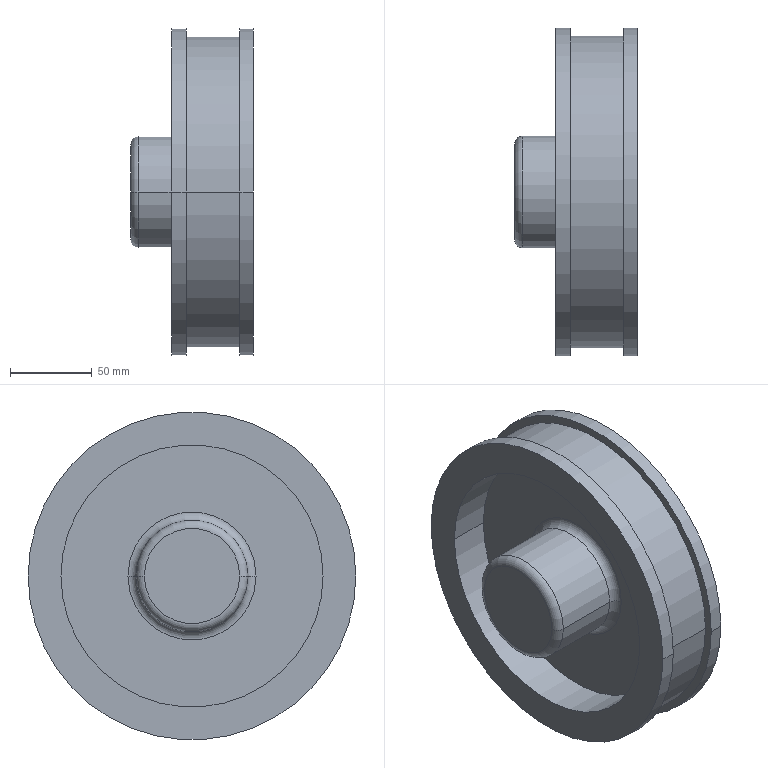Component | SolidWorks | AxisHead-1 | 1 solid | 23 faces | box 75 x 200 x 200 mm | volume 949663 mm3 | cylinder 12 | plane 7 | torus 4 | commonest cylinder face diameters 200 x4 160 x4 190 x2 68.235 x2
build123d program:
from build123d import *


with BuildPart() as part:
    # Sketch1 → Revolve1 (revolve)
    with BuildSketch(Plane.XZ, mode=Mode.PRIVATE) as revolve1_sk:
        with BuildLine():
            Line((80, 0.4717), (0, 0.4717))
            Line((0, 0.4717), (0, -64.528))
            Line((0, -64.528), (29.118, -64.528))
            ThreePointArc((29.118, -64.528), (32.653, -63.064), (34.118, -59.528))
            Line((34.118, -59.528), (34.118, -19.528))
            ThreePointArc((34.118, -19.528), (35.582, -15.993), (39.118, -14.528))
            Line((39.118, -14.528), (80, -14.528))
            Line((80, -14.528), (80, -39.528))
            Line((80, -39.528), (100, -39.528))
            Line((100, -39.528), (100, -30.551))
            Line((100, -30.551), (95, -30.551))
            Line((95, -30.551), (95, 2.206))
            Line((95, 2.206), (100, 2.206))
            Line((100, 2.206), (100, 10.472))
            Line((100, 10.472), (80, 10.472))
            Line((80, 10.472), (80, 0.4717))
        make_face()
    revolve(revolve1_sk.sketch.rotate(Axis((0, 0, 10.472), (0, 0, -1)), 180), axis=Axis((0, 0, 10.472), (0, 0, -1)))


solid = part.part

# Placed as in the assembly
solid = solid.moved(Location((-779.247, 870.769, 1116.347), (0, 90, 0)))
STEP:
#1=COLOUR_RGB('',0.7922,0.8196,0.9333);
#2=FILL_AREA_STYLE_COLOUR('',#1);
#3=FILL_AREA_STYLE('',(#2));
#4=SURFACE_STYLE_FILL_AREA(#3);
#5=SURFACE_SIDE_STYLE('',(#4));
#6=SURFACE_STYLE_USAGE(.BOTH.,#5);
#7=PRESENTATION_STYLE_ASSIGNMENT((#6));
#8=CARTESIAN_POINT('',(-30.267,30.345,43.951));
#9=VERTEX_POINT('',#8);
#10=CARTESIAN_POINT('',(-30.267,38.219,43.951));
#11=VERTEX_POINT('',#10);
#12=CARTESIAN_POINT('',(-30.267,34.282,43.951));
#13=DIRECTION('',(-1.,0.,0.));
#14=DIRECTION('',(0.,-1.,0.));
#15=AXIS2_PLACEMENT_3D('',#12,#13,#14);
#16=CIRCLE('',#15,3.937);
#17=EDGE_CURVE('',#9,#11,#16,.T.);
#18=ORIENTED_EDGE('',*,*,#17,.T.);
#19=CARTESIAN_POINT('',(-30.592,38.219,43.951));
#20=VERTEX_POINT('',#19);
#21=CARTESIAN_POINT('',(-30.267,38.219,43.951));
#22=DIRECTION('',(-1.,0.,0.));
#23=VECTOR('',#22,39.37);
#24=LINE('',#21,#23);
#25=EDGE_CURVE('',#11,#20,#24,.T.);
#26=ORIENTED_EDGE('',*,*,#25,.T.);
#27=CARTESIAN_POINT('',(-30.592,30.345,43.951));
#28=VERTEX_POINT('',#27);
#29=CARTESIAN_POINT('',(-30.592,34.282,43.951));
#30=DIRECTION('',(-1.,0.,0.));
#31=DIRECTION('',(0.,-1.,0.));
#32=AXIS2_PLACEMENT_3D('',#29,#30,#31);
#33=CIRCLE('',#32,3.937);
#34=EDGE_CURVE('',#28,#20,#33,.T.);
#35=ORIENTED_EDGE('',*,*,#34,.F.);
#36=CARTESIAN_POINT('',(-30.267,30.345,43.951));
#37=DIRECTION('',(-1.,0.,0.));
#38=VECTOR('',#37,39.37);
#39=LINE('',#36,#38);
#40=EDGE_CURVE('',#9,#28,#39,.T.);
#41=ORIENTED_EDGE('',*,*,#40,.F.);
#42=EDGE_LOOP('',(#18,#26,#35,#41));
#43=FACE_OUTER_BOUND('',#42,.T.);
#44=CARTESIAN_POINT('',(-30.267,34.282,43.951));
#45=DIRECTION('',(-1.,0.,0.));
#46=DIRECTION('',(0.,-1.,0.));
#47=AXIS2_PLACEMENT_3D('',#44,#45,#46);
#48=CYLINDRICAL_SURFACE('',#47,3.937);
#49=ADVANCED_FACE('',(#43),#48,.T.);
#50=CARTESIAN_POINT('',(-30.592,30.542,43.951));
#51=VERTEX_POINT('',#50);
#52=CARTESIAN_POINT('',(-30.592,38.022,43.951));
#53=VERTEX_POINT('',#52);
#54=CARTESIAN_POINT('',(-30.592,34.282,43.951));
#55=DIRECTION('',(-1.,0.,0.));
#56=DIRECTION('',(0.,-1.,0.));
#57=AXIS2_PLACEMENT_3D('',#54,#55,#56);
#58=CIRCLE('',#57,3.74);
#59=EDGE_CURVE('',#51,#53,#58,.T.);
#60=ORIENTED_EDGE('',*,*,#59,.T.);
#61=CARTESIAN_POINT('',(-31.882,38.022,43.951));
#62=VERTEX_POINT('',#61);
#63=CARTESIAN_POINT('',(-30.267,38.022,43.951));
#64=DIRECTION('',(-1.,0.,0.));
#65=VECTOR('',#64,39.37);
#66=LINE('',#63,#65);
#67=EDGE_CURVE('',#53,#62,#66,.T.);
#68=ORIENTED_EDGE('',*,*,#67,.T.);
#69=CARTESIAN_POINT('',(-31.882,30.542,43.951));
#70=VERTEX_POINT('',#69);
#71=CARTESIAN_POINT('',(-31.882,34.282,43.951));
#72=DIRECTION('',(-1.,0.,0.));
#73=DIRECTION('',(0.,-1.,0.));
#74=AXIS2_PLACEMENT_3D('',#71,#72,#73);
#75=CIRCLE('',#74,3.74);
#76=EDGE_CURVE('',#70,#62,#75,.T.);
#77=ORIENTED_EDGE('',*,*,#76,.F.);
#78=CARTESIAN_POINT('',(-30.267,30.542,43.951));
#79=DIRECTION('',(-1.,0.,0.));
#80=VECTOR('',#79,39.37);
#81=LINE('',#78,#80);
#82=EDGE_CURVE('',#51,#70,#81,.T.);
#83=ORIENTED_EDGE('',*,*,#82,.F.);
#84=EDGE_LOOP('',(#60,#68,#77,#83));
#85=FACE_OUTER_BOUND('',#84,.T.);
#86=CARTESIAN_POINT('',(-30.267,34.282,43.951));
#87=DIRECTION('',(-1.,0.,0.));
#88=DIRECTION('',(0.,-1.,0.));
#89=AXIS2_PLACEMENT_3D('',#86,#87,#88);
#90=CYLINDRICAL_SURFACE('',#89,3.74);
#91=ADVANCED_FACE('',(#85),#90,.T.);
#92=CARTESIAN_POINT('',(-31.882,30.345,43.951));
#93=VERTEX_POINT('',#92);
#94=CARTESIAN_POINT('',(-31.882,38.219,43.951));
#95=VERTEX_POINT('',#94);
#96=CARTESIAN_POINT('',(-31.882,34.282,43.951));
#97=DIRECTION('',(-1.,0.,0.));
#98=DIRECTION('',(0.,-1.,0.));
#99=AXIS2_PLACEMENT_3D('',#96,#97,#98);
#100=CIRCLE('',#99,3.937);
#101=EDGE_CURVE('',#93,#95,#100,.T.);
#102=ORIENTED_EDGE('',*,*,#101,.T.);
#103=CARTESIAN_POINT('',(-32.235,38.219,43.951));
#104=VERTEX_POINT('',#103);
#105=CARTESIAN_POINT('',(-30.267,38.219,43.951));
#106=DIRECTION('',(-1.,0.,0.));
#107=VECTOR('',#106,39.37);
#108=LINE('',#105,#107);
#109=EDGE_CURVE('',#95,#104,#108,.T.);
#110=ORIENTED_EDGE('',*,*,#109,.T.);
#111=CARTESIAN_POINT('',(-32.235,30.345,43.951));
#112=VERTEX_POINT('',#111);
#113=CARTESIAN_POINT('',(-32.235,34.282,43.951));
#114=DIRECTION('',(-1.,0.,0.));
#115=DIRECTION('',(0.,-1.,0.));
#116=AXIS2_PLACEMENT_3D('',#113,#114,#115);
#117=CIRCLE('',#116,3.937);
#118=EDGE_CURVE('',#112,#104,#117,.T.);
#119=ORIENTED_EDGE('',*,*,#118,.F.);
#120=CARTESIAN_POINT('',(-30.267,30.345,43.951));
#121=DIRECTION('',(-1.,0.,0.));
#122=VECTOR('',#121,39.37);
#123=LINE('',#120,#122);
#124=EDGE_CURVE('',#93,#112,#123,.T.);
#125=ORIENTED_EDGE('',*,*,#124,.F.);
#126=EDGE_LOOP('',(#102,#110,#119,#125));
#127=FACE_OUTER_BOUND('',#126,.T.);
#128=CARTESIAN_POINT('',(-30.267,34.282,43.951));
#129=DIRECTION('',(-1.,0.,0.));
#130=DIRECTION('',(0.,-1.,0.));
#131=AXIS2_PLACEMENT_3D('',#128,#129,#130);
#132=CYLINDRICAL_SURFACE('',#131,3.937);
#133=ADVANCED_FACE('',(#127),#132,.T.);
#134=CARTESIAN_POINT('',(-31.251,37.432,43.951));
#135=VERTEX_POINT('',#134);
#136=CARTESIAN_POINT('',(-31.251,31.133,43.951));
#137=VERTEX_POINT('',#136);
#138=CARTESIAN_POINT('',(-31.251,34.282,43.951));
#139=DIRECTION('',(-1.,0.,0.));
#140=DIRECTION('',(0.,-1.,0.));
#141=AXIS2_PLACEMENT_3D('',#138,#139,#140);
#142=CIRCLE('',#141,3.15);
#143=EDGE_CURVE('',#135,#137,#142,.T.);
#144=ORIENTED_EDGE('',*,*,#143,.F.);
#145=CARTESIAN_POINT('',(-32.235,37.432,43.951));
#146=VERTEX_POINT('',#145);
#147=CARTESIAN_POINT('',(-30.267,37.432,43.951));
#148=DIRECTION('',(-1.,0.,0.));
#149=VECTOR('',#148,39.37);
#150=LINE('',#147,#149);
#151=EDGE_CURVE('',#135,#146,#150,.T.);
#152=ORIENTED_EDGE('',*,*,#151,.T.);
#153=CARTESIAN_POINT('',(-32.235,31.133,43.951));
#154=VERTEX_POINT('',#153);
#155=CARTESIAN_POINT('',(-32.235,34.282,43.951));
#156=DIRECTION('',(-1.,0.,0.));
#157=DIRECTION('',(0.,-1.,0.));
#158=AXIS2_PLACEMENT_3D('',#155,#156,#157);
#159=CIRCLE('',#158,3.15);
#160=EDGE_CURVE('',#146,#154,#159,.T.);
#161=ORIENTED_EDGE('',*,*,#160,.T.);
#162=CARTESIAN_POINT('',(-30.267,31.133,43.951));
#163=DIRECTION('',(-1.,0.,0.));
#164=VECTOR('',#163,39.37);
#165=LINE('',#162,#164);
#166=EDGE_CURVE('',#137,#154,#165,.T.);
#167=ORIENTED_EDGE('',*,*,#166,.F.);
#168=EDGE_LOOP('',(#144,#152,#161,#167));
#169=FACE_OUTER_BOUND('',#168,.T.);
#170=CARTESIAN_POINT('',(-30.267,34.282,43.951));
#171=DIRECTION('',(-1.,0.,0.));
#172=DIRECTION('',(0.,-1.,0.));
#173=AXIS2_PLACEMENT_3D('',#170,#171,#172);
#174=CYLINDRICAL_SURFACE('',#173,3.15);
#175=ADVANCED_FACE('',(#169),#174,.F.);
#176=CARTESIAN_POINT('',(-31.448,35.625,43.951));
#177=VERTEX_POINT('',#176);
#178=CARTESIAN_POINT('',(-31.448,32.939,43.951));
#179=VERTEX_POINT('',#178);
#180=CARTESIAN_POINT('',(-31.448,34.282,43.951));
#181=DIRECTION('',(-1.,0.,0.));
#182=DIRECTION('',(0.,-1.,0.));
#183=AXIS2_PLACEMENT_3D('',#180,#181,#182);
#184=CIRCLE('',#183,1.343);
#185=EDGE_CURVE('',#177,#179,#184,.T.);
#186=ORIENTED_EDGE('',*,*,#185,.F.);
#187=CARTESIAN_POINT('',(-31.251,35.822,43.951));
#188=VERTEX_POINT('',#187);
#189=CARTESIAN_POINT('',(-31.448,35.822,43.951));
#190=DIRECTION('',(0.,-0.,1.));
#191=DIRECTION('',(0.,-1.,0.));
#192=AXIS2_PLACEMENT_3D('',#189,#190,#191);
#193=CIRCLE('',#192,0.1969);
#194=EDGE_CURVE('',#177,#188,#193,.T.);
#195=ORIENTED_EDGE('',*,*,#194,.T.);
#196=CARTESIAN_POINT('',(-31.251,32.742,43.951));
#197=VERTEX_POINT('',#196);
#198=CARTESIAN_POINT('',(-31.251,34.282,43.951));
#199=DIRECTION('',(-1.,0.,0.));
#200=DIRECTION('',(0.,-1.,0.));
#201=AXIS2_PLACEMENT_3D('',#198,#199,#200);
#202=CIRCLE('',#201,1.54);
#203=EDGE_CURVE('',#188,#197,#202,.T.);
#204=ORIENTED_EDGE('',*,*,#203,.T.);
#205=CARTESIAN_POINT('',(-31.448,32.742,43.951));
#206=DIRECTION('',(0.,0.,-1.));
#207=DIRECTION('',(-1.,0.,0.));
#208=AXIS2_PLACEMENT_3D('',#205,#206,#207);
#209=CIRCLE('',#208,0.1969);
#210=EDGE_CURVE('',#179,#197,#209,.T.);
#211=ORIENTED_EDGE('',*,*,#210,.F.);
#212=EDGE_LOOP('',(#186,#195,#204,#211));
#213=FACE_OUTER_BOUND('',#212,.T.);
#214=CARTESIAN_POINT('',(-31.448,34.282,43.951));
#215=DIRECTION('',(-1.,0.,0.));
#216=DIRECTION('',(0.,-1.,0.));
#217=AXIS2_PLACEMENT_3D('',#214,#215,#216);
#218=TOROIDAL_SURFACE('',#217,1.54,0.1969);
#219=ADVANCED_FACE('',(#213),#218,.F.);
#220=CARTESIAN_POINT('',(-31.448,34.282,43.951));
#221=DIRECTION('',(-1.,0.,0.));
#222=DIRECTION('',(0.,-1.,0.));
#223=AXIS2_PLACEMENT_3D('',#220,#221,#222);
#224=CIRCLE('',#223,1.343);
#225=EDGE_CURVE('',#179,#177,#224,.T.);
#226=ORIENTED_EDGE('',*,*,#225,.T.);
#227=CARTESIAN_POINT('',(-33.023,35.625,43.951));
#228=VERTEX_POINT('',#227);
#229=CARTESIAN_POINT('',(-30.267,35.625,43.951));
#230=DIRECTION('',(-1.,0.,0.));
#231=VECTOR('',#230,39.37);
#232=LINE('',#229,#231);
#233=EDGE_CURVE('',#177,#228,#232,.T.);
#234=ORIENTED_EDGE('',*,*,#233,.T.);
#235=CARTESIAN_POINT('',(-33.023,32.939,43.951));
#236=VERTEX_POINT('',#235);
#237=CARTESIAN_POINT('',(-33.023,34.282,43.951));
#238=DIRECTION('',(-1.,0.,0.));
#239=DIRECTION('',(0.,-1.,0.));
#240=AXIS2_PLACEMENT_3D('',#237,#238,#239);
#241=CIRCLE('',#240,1.343);
#242=EDGE_CURVE('',#236,#228,#241,.T.);
#243=ORIENTED_EDGE('',*,*,#242,.F.);
#244=CARTESIAN_POINT('',(-30.267,32.939,43.951));
#245=DIRECTION('',(-1.,0.,0.));
#246=VECTOR('',#245,39.37);
#247=LINE('',#244,#246);
#248=EDGE_CURVE('',#179,#236,#247,.T.);
#249=ORIENTED_EDGE('',*,*,#248,.F.);
#250=EDGE_LOOP('',(#226,#234,#243,#249));
#251=FACE_OUTER_BOUND('',#250,.T.);
#252=CARTESIAN_POINT('',(-30.267,34.282,43.951));
#253=DIRECTION('',(-1.,0.,0.));
#254=DIRECTION('',(0.,-1.,0.));
#255=AXIS2_PLACEMENT_3D('',#252,#253,#254);
#256=CYLINDRICAL_SURFACE('',#255,1.343);
#257=ADVANCED_FACE('',(#251),#256,.T.);
#258=ORIENTED_EDGE('',*,*,#242,.T.);
#259=CARTESIAN_POINT('',(-33.219,35.429,43.951));
#260=VERTEX_POINT('',#259);
#261=CARTESIAN_POINT('',(-33.023,35.429,43.951));
#262=DIRECTION('',(0.,-0.,1.));
#263=DIRECTION('',(0.,-1.,0.));
#264=AXIS2_PLACEMENT_3D('',#261,#262,#263);
#265=CIRCLE('',#264,0.1969);
#266=EDGE_CURVE('',#228,#260,#265,.T.);
#267=ORIENTED_EDGE('',*,*,#266,.T.);
#268=CARTESIAN_POINT('',(-33.219,33.136,43.951));
#269=VERTEX_POINT('',#268);
#270=CARTESIAN_POINT('',(-33.219,34.282,43.951));
#271=DIRECTION('',(-1.,0.,0.));
#272=DIRECTION('',(0.,-1.,0.));
#273=AXIS2_PLACEMENT_3D('',#270,#271,#272);
#274=CIRCLE('',#273,1.146);
#275=EDGE_CURVE('',#269,#260,#274,.T.);
#276=ORIENTED_EDGE('',*,*,#275,.F.);
#277=CARTESIAN_POINT('',(-33.023,33.136,43.951));
#278=DIRECTION('',(0.,0.,-1.));
#279=DIRECTION('',(-1.,0.,0.));
#280=AXIS2_PLACEMENT_3D('',#277,#278,#279);
#281=CIRCLE('',#280,0.1969);
#282=EDGE_CURVE('',#236,#269,#281,.T.);
#283=ORIENTED_EDGE('',*,*,#282,.F.);
#284=EDGE_LOOP('',(#258,#267,#276,#283));
#285=FACE_OUTER_BOUND('',#284,.T.);
#286=CARTESIAN_POINT('',(-33.023,34.282,43.951));
#287=DIRECTION('',(-1.,0.,0.));
#288=DIRECTION('',(0.,-1.,0.));
#289=AXIS2_PLACEMENT_3D('',#286,#287,#288);
#290=TOROIDAL_SURFACE('',#289,1.146,0.1969);
#291=ADVANCED_FACE('',(#285),#290,.T.);
#292=CARTESIAN_POINT('',(-30.267,37.432,43.951));
#293=VERTEX_POINT('',#292);
#294=CARTESIAN_POINT('',(-30.267,31.133,43.951));
#295=VERTEX_POINT('',#294);
#296=CARTESIAN_POINT('',(-30.267,34.282,43.951));
#297=DIRECTION('',(-1.,0.,0.));
#298=DIRECTION('',(0.,-1.,0.));
#299=AXIS2_PLACEMENT_3D('',#296,#297,#298);
#300=CIRCLE('',#299,3.15);
#301=EDGE_CURVE('',#293,#295,#300,.T.);
#302=ORIENTED_EDGE('',*,*,#301,.F.);
#303=CARTESIAN_POINT('',(-30.66,37.432,43.951));
#304=VERTEX_POINT('',#303);
#305=CARTESIAN_POINT('',(-30.267,37.432,43.951));
#306=DIRECTION('',(-1.,0.,0.));
#307=VECTOR('',#306,39.37);
#308=LINE('',#305,#307);
#309=EDGE_CURVE('',#293,#304,#308,.T.);
#310=ORIENTED_EDGE('',*,*,#309,.T.);
#311=CARTESIAN_POINT('',(-30.66,31.133,43.951));
#312=VERTEX_POINT('',#311);
#313=CARTESIAN_POINT('',(-30.66,34.282,43.951));
#314=DIRECTION('',(-1.,0.,0.));
#315=DIRECTION('',(0.,-1.,0.));
#316=AXIS2_PLACEMENT_3D('',#313,#314,#315);
#317=CIRCLE('',#316,3.15);
#318=EDGE_CURVE('',#304,#312,#317,.T.);
#319=ORIENTED_EDGE('',*,*,#318,.T.);
#320=CARTESIAN_POINT('',(-30.267,31.133,43.951));
#321=DIRECTION('',(-1.,0.,0.));
#322=VECTOR('',#321,39.37);
#323=LINE('',#320,#322);
#324=EDGE_CURVE('',#295,#312,#323,.T.);
#325=ORIENTED_EDGE('',*,*,#324,.F.);
#326=EDGE_LOOP('',(#302,#310,#319,#325));
#327=FACE_OUTER_BOUND('',#326,.T.);
#328=CARTESIAN_POINT('',(-30.267,34.282,43.951));
#329=DIRECTION('',(-1.,0.,0.));
#330=DIRECTION('',(0.,-1.,0.));
#331=AXIS2_PLACEMENT_3D('',#328,#329,#330);
#332=CYLINDRICAL_SURFACE('',#331,3.15);
#333=ADVANCED_FACE('',(#327),#332,.F.);
#334=ORIENTED_EDGE('',*,*,#309,.F.);
#335=CARTESIAN_POINT('',(-30.267,34.282,43.951));
#336=DIRECTION('',(-1.,0.,0.));
#337=DIRECTION('',(0.,-1.,0.));
#338=AXIS2_PLACEMENT_3D('',#335,#336,#337);
#339=CIRCLE('',#338,3.15);
#340=EDGE_CURVE('',#295,#293,#339,.T.);
#341=ORIENTED_EDGE('',*,*,#340,.F.);
#342=ORIENTED_EDGE('',*,*,#324,.T.);
#343=CARTESIAN_POINT('',(-30.66,34.282,43.951));
#344=DIRECTION('',(-1.,0.,0.));
#345=DIRECTION('',(0.,-1.,0.));
#346=AXIS2_PLACEMENT_3D('',#343,#344,#345);
#347=CIRCLE('',#346,3.15);
#348=EDGE_CURVE('',#312,#304,#347,.T.);
#349=ORIENTED_EDGE('',*,*,#348,.T.);
#350=EDGE_LOOP('',(#334,#341,#342,#349));
#351=FACE_OUTER_BOUND('',#350,.T.);
#352=CARTESIAN_POINT('',(-30.267,34.282,43.951));
#353=DIRECTION('',(-1.,0.,0.));
#354=DIRECTION('',(0.,-1.,0.));
#355=AXIS2_PLACEMENT_3D('',#352,#353,#354);
#356=CYLINDRICAL_SURFACE('',#355,3.15);
#357=ADVANCED_FACE('',(#351),#356,.F.);
#358=ORIENTED_EDGE('',*,*,#348,.F.);
#359=ORIENTED_EDGE('',*,*,#318,.F.);
#360=EDGE_LOOP('',(#358,#359));
#361=FACE_OUTER_BOUND('',#360,.T.);
#362=CARTESIAN_POINT('',(-30.66,37.432,43.951));
#363=DIRECTION('',(1.,0.,0.));
#364=DIRECTION('',(0.,1.,0.));
#365=AXIS2_PLACEMENT_3D('',#362,#363,#364);
#366=PLANE('',#365);
#367=ADVANCED_FACE('',(#361),#366,.T.);
#368=ORIENTED_EDGE('',*,*,#275,.T.);
#369=CARTESIAN_POINT('',(-33.219,34.282,43.951));
#370=DIRECTION('',(-1.,0.,0.));
#371=DIRECTION('',(0.,-1.,0.));
#372=AXIS2_PLACEMENT_3D('',#369,#370,#371);
#373=CIRCLE('',#372,1.146);
#374=EDGE_CURVE('',#260,#269,#373,.T.);
#375=ORIENTED_EDGE('',*,*,#374,.T.);
#376=EDGE_LOOP('',(#368,#375));
#377=FACE_OUTER_BOUND('',#376,.T.);
#378=CARTESIAN_POINT('',(-33.219,34.282,43.951));
#379=DIRECTION('',(-1.,0.,0.));
#380=DIRECTION('',(0.,-1.,0.));
#381=AXIS2_PLACEMENT_3D('',#378,#379,#380);
#382=PLANE('',#381);
#383=ADVANCED_FACE('',(#377),#382,.T.);
#384=ORIENTED_EDGE('',*,*,#266,.F.);
#385=CARTESIAN_POINT('',(-33.023,34.282,43.951));
#386=DIRECTION('',(-1.,0.,0.));
#387=DIRECTION('',(0.,-1.,0.));
#388=AXIS2_PLACEMENT_3D('',#385,#386,#387);
#389=CIRCLE('',#388,1.343);
#390=EDGE_CURVE('',#228,#236,#389,.T.);
#391=ORIENTED_EDGE('',*,*,#390,.T.);
#392=ORIENTED_EDGE('',*,*,#282,.T.);
#393=ORIENTED_EDGE('',*,*,#374,.F.);
#394=EDGE_LOOP('',(#384,#391,#392,#393));
#395=FACE_OUTER_BOUND('',#394,.T.);
#396=CARTESIAN_POINT('',(-33.023,34.282,43.951));
#397=DIRECTION('',(-1.,0.,0.));
#398=DIRECTION('',(0.,-1.,0.));
#399=AXIS2_PLACEMENT_3D('',#396,#397,#398);
#400=TOROIDAL_SURFACE('',#399,1.146,0.1969);
#401=ADVANCED_FACE('',(#395),#400,.T.);
#402=ORIENTED_EDGE('',*,*,#233,.F.);
#403=ORIENTED_EDGE('',*,*,#185,.T.);
#404=ORIENTED_EDGE('',*,*,#248,.T.);
#405=ORIENTED_EDGE('',*,*,#390,.F.);
#406=EDGE_LOOP('',(#402,#403,#404,#405));
#407=FACE_OUTER_BOUND('',#406,.T.);
#408=CARTESIAN_POINT('',(-30.267,34.282,43.951));
#409=DIRECTION('',(-1.,0.,0.));
#410=DIRECTION('',(0.,-1.,0.));
#411=AXIS2_PLACEMENT_3D('',#408,#409,#410);
#412=CYLINDRICAL_SURFACE('',#411,1.343);
#413=ADVANCED_FACE('',(#407),#412,.T.);
#414=ORIENTED_EDGE('',*,*,#194,.F.);
#415=ORIENTED_EDGE('',*,*,#225,.F.);
#416=ORIENTED_EDGE('',*,*,#210,.T.);
#417=CARTESIAN_POINT('',(-31.251,34.282,43.951));
#418=DIRECTION('',(-1.,0.,0.));
#419=DIRECTION('',(0.,-1.,0.));
#420=AXIS2_PLACEMENT_3D('',#417,#418,#419);
#421=CIRCLE('',#420,1.54);
#422=EDGE_CURVE('',#197,#188,#421,.T.);
#423=ORIENTED_EDGE('',*,*,#422,.T.);
#424=EDGE_LOOP('',(#414,#415,#416,#423));
#425=FACE_OUTER_BOUND('',#424,.T.);
#426=CARTESIAN_POINT('',(-31.448,34.282,43.951));
#427=DIRECTION('',(-1.,0.,0.));
#428=DIRECTION('',(0.,-1.,0.));
#429=AXIS2_PLACEMENT_3D('',#426,#427,#428);
#430=TOROIDAL_SURFACE('',#429,1.54,0.1969);
#431=ADVANCED_FACE('',(#425),#430,.F.);
#432=CARTESIAN_POINT('',(-31.251,34.282,43.951));
#433=DIRECTION('',(-1.,0.,0.));
#434=DIRECTION('',(0.,-1.,0.));
#435=AXIS2_PLACEMENT_3D('',#432,#433,#434);
#436=CIRCLE('',#435,3.15);
#437=EDGE_CURVE('',#137,#135,#436,.T.);
#438=ORIENTED_EDGE('',*,*,#437,.T.);
#439=ORIENTED_EDGE('',*,*,#143,.T.);
#440=EDGE_LOOP('',(#438,#439));
#441=FACE_OUTER_BOUND('',#440,.T.);
#442=ORIENTED_EDGE('',*,*,#422,.F.);
#443=ORIENTED_EDGE('',*,*,#203,.F.);
#444=EDGE_LOOP('',(#442,#443));
#445=FACE_BOUND('',#444,.T.);
#446=CARTESIAN_POINT('',(-31.251,35.822,43.951));
#447=DIRECTION('',(-1.,0.,0.));
#448=DIRECTION('',(0.,-1.,0.));
#449=AXIS2_PLACEMENT_3D('',#446,#447,#448);
#450=PLANE('',#449);
#451=ADVANCED_FACE('',(#441,#445),#450,.T.);
#452=ORIENTED_EDGE('',*,*,#151,.F.);
#453=ORIENTED_EDGE('',*,*,#437,.F.);
#454=ORIENTED_EDGE('',*,*,#166,.T.);
#455=CARTESIAN_POINT('',(-32.235,34.282,43.951));
#456=DIRECTION('',(-1.,0.,0.));
#457=DIRECTION('',(0.,-1.,0.));
#458=AXIS2_PLACEMENT_3D('',#455,#456,#457);
#459=CIRCLE('',#458,3.15);
#460=EDGE_CURVE('',#154,#146,#459,.T.);
#461=ORIENTED_EDGE('',*,*,#460,.T.);
#462=EDGE_LOOP('',(#452,#453,#454,#461));
#463=FACE_OUTER_BOUND('',#462,.T.);
#464=CARTESIAN_POINT('',(-30.267,34.282,43.951));
#465=DIRECTION('',(-1.,0.,0.));
#466=DIRECTION('',(0.,-1.,0.));
#467=AXIS2_PLACEMENT_3D('',#464,#465,#466);
#468=CYLINDRICAL_SURFACE('',#467,3.15);
#469=ADVANCED_FACE('',(#463),#468,.F.);
#470=ORIENTED_EDGE('',*,*,#118,.T.);
#471=CARTESIAN_POINT('',(-32.235,34.282,43.951));
#472=DIRECTION('',(-1.,0.,0.));
#473=DIRECTION('',(0.,-1.,0.));
#474=AXIS2_PLACEMENT_3D('',#471,#472,#473);
#475=CIRCLE('',#474,3.937);
#476=EDGE_CURVE('',#104,#112,#475,.T.);
#477=ORIENTED_EDGE('',*,*,#476,.T.);
#478=EDGE_LOOP('',(#470,#477));
#479=FACE_OUTER_BOUND('',#478,.T.);
#480=ORIENTED_EDGE('',*,*,#460,.F.);
#481=ORIENTED_EDGE('',*,*,#160,.F.);
#482=EDGE_LOOP('',(#480,#481));
#483=FACE_BOUND('',#482,.T.);
#484=CARTESIAN_POINT('',(-32.235,37.432,43.951));
#485=DIRECTION('',(-1.,0.,0.));
#486=DIRECTION('',(0.,-1.,0.));
#487=AXIS2_PLACEMENT_3D('',#484,#485,#486);
#488=PLANE('',#487);
#489=ADVANCED_FACE('',(#479,#483),#488,.T.);
#490=ORIENTED_EDGE('',*,*,#109,.F.);
#491=CARTESIAN_POINT('',(-31.882,34.282,43.951));
#492=DIRECTION('',(-1.,0.,0.));
#493=DIRECTION('',(0.,-1.,0.));
#494=AXIS2_PLACEMENT_3D('',#491,#492,#493);
#495=CIRCLE('',#494,3.937);
#496=EDGE_CURVE('',#95,#93,#495,.T.);
#497=ORIENTED_EDGE('',*,*,#496,.T.);
#498=ORIENTED_EDGE('',*,*,#124,.T.);
#499=ORIENTED_EDGE('',*,*,#476,.F.);
#500=EDGE_LOOP('',(#490,#497,#498,#499));
#501=FACE_OUTER_BOUND('',#500,.T.);
#502=CARTESIAN_POINT('',(-30.267,34.282,43.951));
#503=DIRECTION('',(-1.,0.,0.));
#504=DIRECTION('',(0.,-1.,0.));
#505=AXIS2_PLACEMENT_3D('',#502,#503,#504);
#506=CYLINDRICAL_SURFACE('',#505,3.937);
#507=ADVANCED_FACE('',(#501),#506,.T.);
#508=ORIENTED_EDGE('',*,*,#76,.T.);
#509=CARTESIAN_POINT('',(-31.882,34.282,43.951));
#510=DIRECTION('',(-1.,0.,0.));
#511=DIRECTION('',(0.,-1.,0.));
#512=AXIS2_PLACEMENT_3D('',#509,#510,#511);
#513=CIRCLE('',#512,3.74);
#514=EDGE_CURVE('',#62,#70,#513,.T.);
#515=ORIENTED_EDGE('',*,*,#514,.T.);
#516=EDGE_LOOP('',(#508,#515));
#517=FACE_BOUND('',#516,.T.);
#518=ORIENTED_EDGE('',*,*,#101,.F.);
#519=ORIENTED_EDGE('',*,*,#496,.F.);
#520=EDGE_LOOP('',(#518,#519));
#521=FACE_OUTER_BOUND('',#520,.T.);
#522=CARTESIAN_POINT('',(-31.882,38.219,43.951));
#523=DIRECTION('',(1.,0.,0.));
#524=DIRECTION('',(0.,1.,0.));
#525=AXIS2_PLACEMENT_3D('',#522,#523,#524);
#526=PLANE('',#525);
#527=ADVANCED_FACE('',(#517,#521),#526,.T.);
#528=ORIENTED_EDGE('',*,*,#67,.F.);
#529=CARTESIAN_POINT('',(-30.592,34.282,43.951));
#530=DIRECTION('',(-1.,0.,0.));
#531=DIRECTION('',(0.,-1.,0.));
#532=AXIS2_PLACEMENT_3D('',#529,#530,#531);
#533=CIRCLE('',#532,3.74);
#534=EDGE_CURVE('',#53,#51,#533,.T.);
#535=ORIENTED_EDGE('',*,*,#534,.T.);
#536=ORIENTED_EDGE('',*,*,#82,.T.);
#537=ORIENTED_EDGE('',*,*,#514,.F.);
#538=EDGE_LOOP('',(#528,#535,#536,#537));
#539=FACE_OUTER_BOUND('',#538,.T.);
#540=CARTESIAN_POINT('',(-30.267,34.282,43.951));
#541=DIRECTION('',(-1.,0.,0.));
#542=DIRECTION('',(0.,-1.,0.));
#543=AXIS2_PLACEMENT_3D('',#540,#541,#542);
#544=CYLINDRICAL_SURFACE('',#543,3.74);
#545=ADVANCED_FACE('',(#539),#544,.T.);
#546=ORIENTED_EDGE('',*,*,#34,.T.);
#547=CARTESIAN_POINT('',(-30.592,34.282,43.951));
#548=DIRECTION('',(-1.,0.,0.));
#549=DIRECTION('',(0.,-1.,0.));
#550=AXIS2_PLACEMENT_3D('',#547,#548,#549);
#551=CIRCLE('',#550,3.937);
#552=EDGE_CURVE('',#20,#28,#551,.T.);
#553=ORIENTED_EDGE('',*,*,#552,.T.);
#554=EDGE_LOOP('',(#546,#553));
#555=FACE_OUTER_BOUND('',#554,.T.);
#556=ORIENTED_EDGE('',*,*,#59,.F.);
#557=ORIENTED_EDGE('',*,*,#534,.F.);
#558=EDGE_LOOP('',(#556,#557));
#559=FACE_BOUND('',#558,.T.);
#560=CARTESIAN_POINT('',(-30.592,38.022,43.951));
#561=DIRECTION('',(-1.,0.,0.));
#562=DIRECTION('',(0.,-1.,0.));
#563=AXIS2_PLACEMENT_3D('',#560,#561,#562);
#564=PLANE('',#563);
#565=ADVANCED_FACE('',(#555,#559),#564,.T.);
#566=ORIENTED_EDGE('',*,*,#25,.F.);
#567=CARTESIAN_POINT('',(-30.267,34.282,43.951));
#568=DIRECTION('',(-1.,0.,0.));
#569=DIRECTION('',(0.,-1.,0.));
#570=AXIS2_PLACEMENT_3D('',#567,#568,#569);
#571=CIRCLE('',#570,3.937);
#572=EDGE_CURVE('',#11,#9,#571,.T.);
#573=ORIENTED_EDGE('',*,*,#572,.T.);
#574=ORIENTED_EDGE('',*,*,#40,.T.);
#575=ORIENTED_EDGE('',*,*,#552,.F.);
#576=EDGE_LOOP('',(#566,#573,#574,#575));
#577=FACE_OUTER_BOUND('',#576,.T.);
#578=CARTESIAN_POINT('',(-30.267,34.282,43.951));
#579=DIRECTION('',(-1.,0.,0.));
#580=DIRECTION('',(0.,-1.,0.));
#581=AXIS2_PLACEMENT_3D('',#578,#579,#580);
#582=CYLINDRICAL_SURFACE('',#581,3.937);
#583=ADVANCED_FACE('',(#577),#582,.T.);
#584=ORIENTED_EDGE('',*,*,#340,.T.);
#585=ORIENTED_EDGE('',*,*,#301,.T.);
#586=EDGE_LOOP('',(#584,#585));
#587=FACE_BOUND('',#586,.T.);
#588=ORIENTED_EDGE('',*,*,#17,.F.);
#589=ORIENTED_EDGE('',*,*,#572,.F.);
#590=EDGE_LOOP('',(#588,#589));
#591=FACE_OUTER_BOUND('',#590,.T.);
#592=CARTESIAN_POINT('',(-30.267,38.219,43.951));
#593=DIRECTION('',(1.,0.,0.));
#594=DIRECTION('',(0.,1.,0.));
#595=AXIS2_PLACEMENT_3D('',#592,#593,#594);
#596=PLANE('',#595);
#597=ADVANCED_FACE('',(#587,#591),#596,.T.);
#598=CLOSED_SHELL('',(#49,#91,#133,#175,#219,#257,#291,#333,#357,#367,#383,#401,#413,#431,#451,#469,#489,#507,#527,#545,#565,#583,#597));
#599=MANIFOLD_SOLID_BREP('',#598);
#600=STYLED_ITEM('',(#7),#599);
#601=(LENGTH_UNIT()NAMED_UNIT(*)SI_UNIT($,.METRE.));
#602=LENGTH_MEASURE_WITH_UNIT(LENGTH_MEASURE(0.0254),#601);
#603=DIMENSIONAL_EXPONENTS(1.,0.,0.,0.,0.,0.,0.);
#604=(CONVERSION_BASED_UNIT('',#602)LENGTH_UNIT()NAMED_UNIT(#603));
#605=UNCERTAINTY_MEASURE_WITH_UNIT(LENGTH_MEASURE(0.00001),#604,'','');
#606=(NAMED_UNIT(*)PLANE_ANGLE_UNIT()SI_UNIT($,.RADIAN.));
#607=(NAMED_UNIT(*)SI_UNIT($,.STERADIAN.)SOLID_ANGLE_UNIT());
#608=(GEOMETRIC_REPRESENTATION_CONTEXT(3)GLOBAL_UNCERTAINTY_ASSIGNED_CONTEXT((#605))GLOBAL_UNIT_ASSIGNED_CONTEXT((#604,#606,#607))REPRESENTATION_CONTEXT('',''));
#609=MECHANICAL_DESIGN_GEOMETRIC_PRESENTATION_REPRESENTATION('',(#600),#608);
#610=PRESENTATION_LAYER_ASSIGNMENT('','',(#600));
#611=CARTESIAN_POINT('',(0.,0.,0.));
#612=DIRECTION('',(0.,0.,1.));
#613=DIRECTION('',(1.,0.,0.));
#614=AXIS2_PLACEMENT_3D('',#611,#612,#613);
#615=(LENGTH_UNIT()NAMED_UNIT(*)SI_UNIT($,.METRE.));
#616=LENGTH_MEASURE_WITH_UNIT(LENGTH_MEASURE(0.0254),#615);
#617=DIMENSIONAL_EXPONENTS(1.,0.,0.,0.,0.,0.,0.);
#618=(CONVERSION_BASED_UNIT('',#616)LENGTH_UNIT()NAMED_UNIT(#617));
#619=UNCERTAINTY_MEASURE_WITH_UNIT(LENGTH_MEASURE(0.00001),#618,'','');
#620=(NAMED_UNIT(*)PLANE_ANGLE_UNIT()SI_UNIT($,.RADIAN.));
#621=(NAMED_UNIT(*)SI_UNIT($,.STERADIAN.)SOLID_ANGLE_UNIT());
#622=(GEOMETRIC_REPRESENTATION_CONTEXT(3)GLOBAL_UNCERTAINTY_ASSIGNED_CONTEXT((#619))GLOBAL_UNIT_ASSIGNED_CONTEXT((#618,#620,#621))REPRESENTATION_CONTEXT('',''));
#623=ADVANCED_BREP_SHAPE_REPRESENTATION('',(#599,#614),#622);